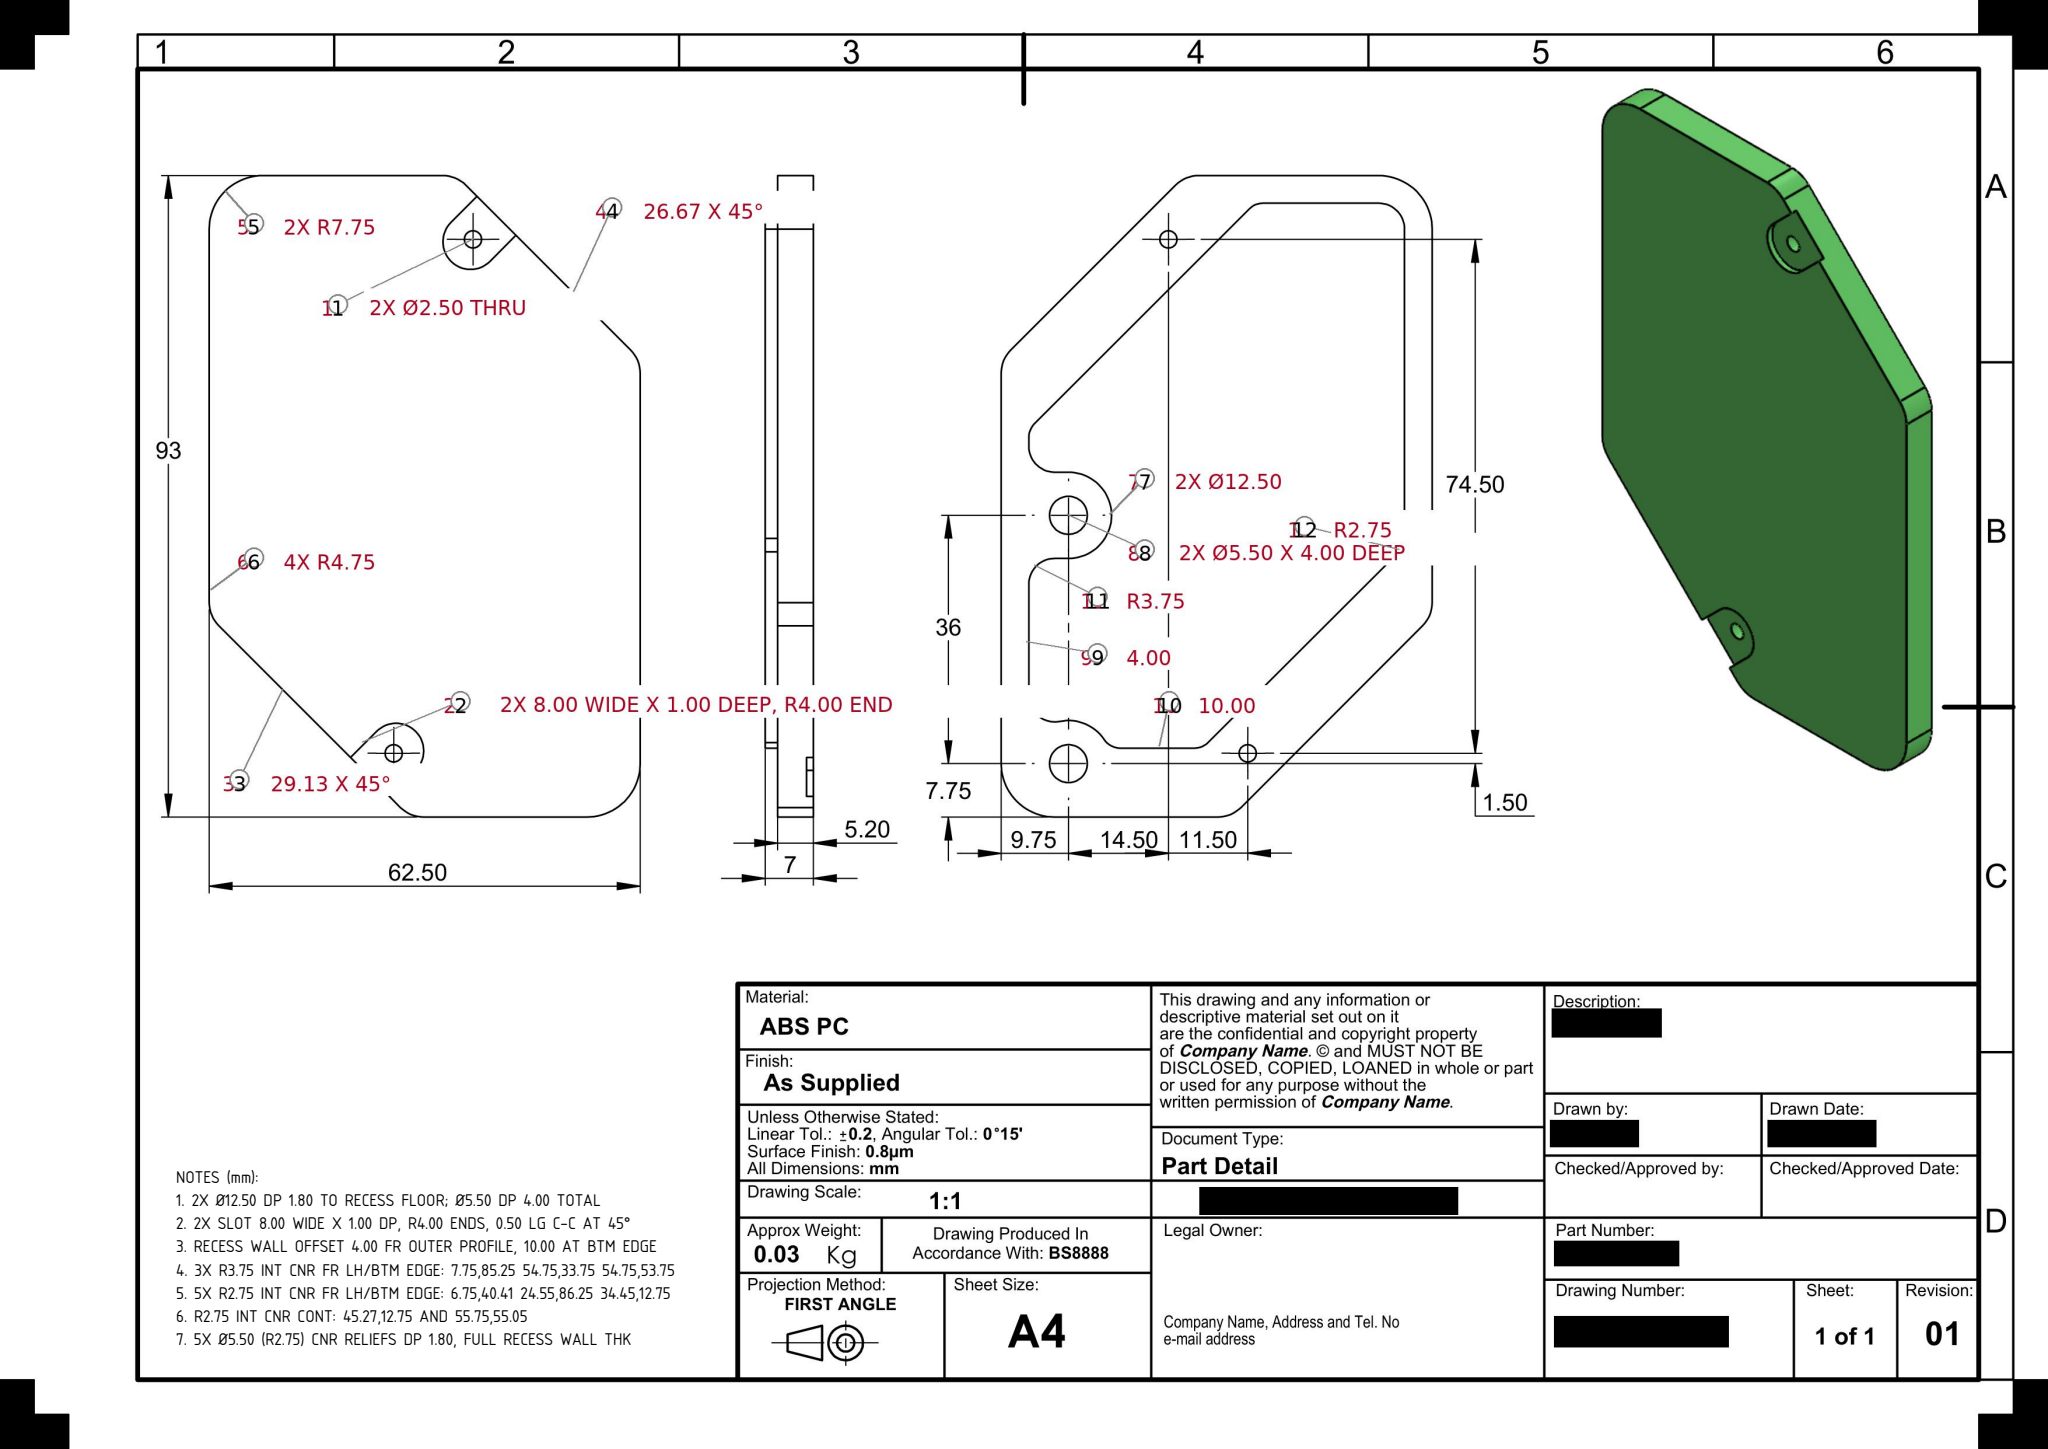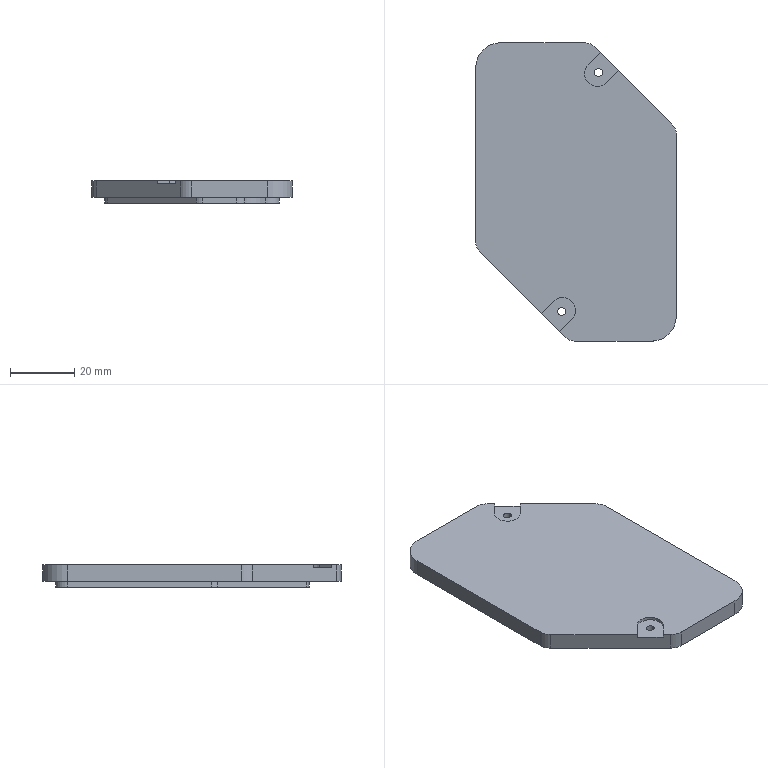Part | SolidWorks | mm | 1 solid | 54 faces | box 62.5 x 93 x 7 mm | volume 31419 mm3 | cylinder 27 | plane 26 | spline 1 | commonest cylinder face diameters 5.5 x9 2.5 x4 9.5 x4 8 x3 7.5 x3 15.5 x2 12.5 x2
Drawing notes:
2X Ø12.50 DP 1.80 TO RECESS FLOOR; Ø5.50 DP 4.00 TOTAL | from the solid: Ø12.50 cyl L=1.80 at (52.75,7.75)&(52.75,43.75); Ø5.50 L=2.20 same axes; floor plane z=1.80 (1.80+2.20=4.00)
2X SLOT 8.00 WIDE X 1.00 DP, R4.00 ENDS, 0.50 LG C-C AT 45° | from the solid: Ø8.0 L=1.0 at (27.10,9.60) vs Ø2.50 at (26.75,9.25) and (37.90,83.40) vs (38.25,83.75): offset 0.35,0.35 = 0.495 at 45°
RECESS WALL OFFSET 4.00 FR OUTER PROFILE, 10.00 AT BTM EDGE | from the solid: planes x=4.0 & x=58.5 (4.00 fr x=0 / x=62.5), y=89.0 (4.00 fr y=93), y=10.0 (10.00 fr y=0); recess dp 7.00-1.80=5.20
3X R3.75 INT CNR FR LH/BTM EDGE: 7.75,85.25 54.75,33.75 54.75,53.75 | from the solid: Ø7.5 cyl L=1.80 at (7.75,85.25),(54.75,33.75),(54.75,53.75)
5X R2.75 INT CNR FR LH/BTM EDGE: 6.75,40.41 24.55,86.25 34.45,12.75 | from the solid: Ø5.5 cyl L=1.80 at (6.75,40.41),(24.55,86.25),(34.45,12.75)
R2.75 INT CNR CONT: 45.27,12.75 AND 55.75,55.05 | from the solid: Ø5.5 cyl L=1.80 at (45.27,12.75),(55.75,55.05)
5X Ø5.50 (R2.75) CNR RELIEFS DP 1.80, FULL RECESS WALL THK | from the solid: Ø5.5 corner cylinders length 1.80 spanning z=0 to z=1.80 floor plane